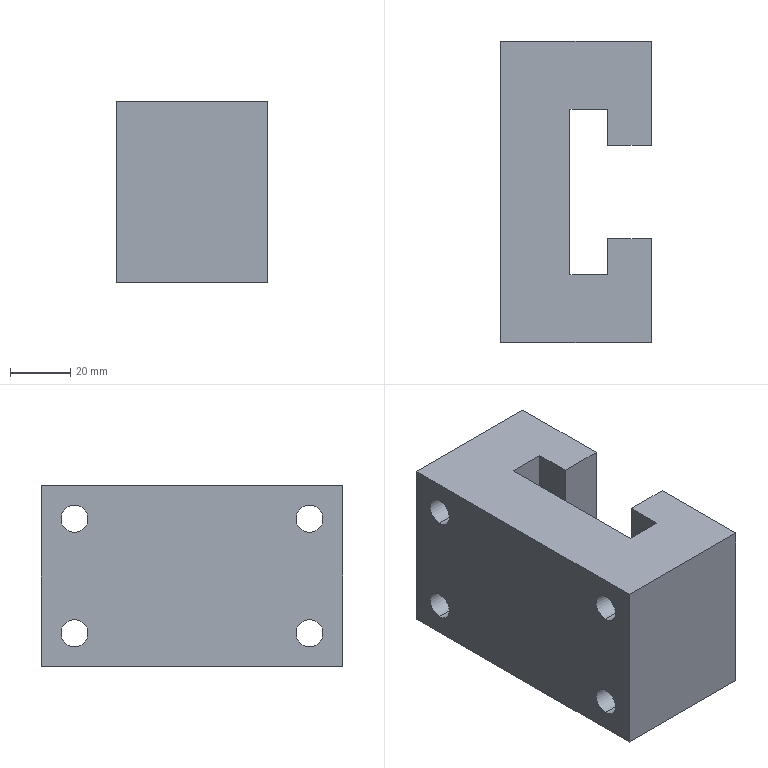Component | SolidWorks | ZN-A-019-1 | 1 solid | 34 faces | box 50 x 100 x 60 mm | volume 215166 mm3 | plane 18 | cylinder 16 | commonest cylinder face diameters 15 x8 9 x8
build123d program:
from build123d import *

# Parameters (mm, degrees)
SKETCH1_W                                       = 100
SKETCH1_H                                       = 50
BOSS_EXTRUDE1_DEPTH                             = 60
CUT_EXTRUDE1_DEPTH                              = 83.006
M8_HEX_SOCKET_HEAD_CAP_SCREW_CBORE1_D           = 9
M8_HEX_SOCKET_HEAD_CAP_SCREW_CBORE1_CBORE_D     = 15
M8_HEX_SOCKET_HEAD_CAP_SCREW_CBORE1_CBORE_DEPTH = 8.6


with BuildPart() as part:
    # Sketch1 → Boss-Extrude1 (new body)
    with BuildSketch(Plane.XY):
        Rectangle(SKETCH1_W, SKETCH1_H)
    extrude(amount=BOSS_EXTRUDE1_DEPTH)

    # Sketch2 → Cut-Extrude1 (cut, through all)
    with BuildSketch(Plane(origin=(0, 0, 0), x_dir=(-1, 0, 0), z_dir=(0, 0, -1))):
        Polygon((-15.5, 25), (15.5, 25), (15.5, 10.5), (27.5, 10.5), (27.5, -2), (-27.5, -2), (-27.5, 10.5), (-15.5, 10.5), align=None)
    extrude(amount=-CUT_EXTRUDE1_DEPTH, mode=Mode.SUBTRACT)

    # M8 Hex Socket Head Cap Screw CBORE1 (through all)
    with Locations(Plane(origin=(0, 25, 0), x_dir=(1, 0, 0), z_dir=(0, 1, 0))):
        with Locations((-39, -11), (-39, -49), (39, -11), (39, -49)):
            CounterBoreHole(M8_HEX_SOCKET_HEAD_CAP_SCREW_CBORE1_D / 2, M8_HEX_SOCKET_HEAD_CAP_SCREW_CBORE1_CBORE_D / 2, M8_HEX_SOCKET_HEAD_CAP_SCREW_CBORE1_CBORE_DEPTH)


solid = part.part

# Placed as in the assembly
solid = solid.moved(Location((540.892, 232.499, 73), (0, 0, -90)))
STEP:
#1=COLOUR_RGB('',0.7922,0.8196,0.9333);
#2=FILL_AREA_STYLE_COLOUR('',#1);
#3=FILL_AREA_STYLE('',(#2));
#4=SURFACE_STYLE_FILL_AREA(#3);
#5=SURFACE_SIDE_STYLE('',(#4));
#6=SURFACE_STYLE_USAGE(.BOTH.,#5);
#7=PRESENTATION_STYLE_ASSIGNMENT((#6));
#8=CARTESIAN_POINT('',(21.941,10.689,3.012));
#9=VERTEX_POINT('',#8);
#10=CARTESIAN_POINT('',(21.941,10.689,3.602));
#11=VERTEX_POINT('',#10);
#12=CARTESIAN_POINT('',(21.941,10.689,3.307));
#13=DIRECTION('',(1.,-0.,0.));
#14=DIRECTION('',(0.,-0.,1.));
#15=AXIS2_PLACEMENT_3D('',#12,#13,#14);
#16=CIRCLE('',#15,0.2953);
#17=EDGE_CURVE('',#9,#11,#16,.T.);
#18=ORIENTED_EDGE('',*,*,#17,.F.);
#19=CARTESIAN_POINT('',(22.279,10.689,3.012));
#20=VERTEX_POINT('',#19);
#21=CARTESIAN_POINT('',(22.279,10.689,3.012));
#22=DIRECTION('',(1.,-0.,0.));
#23=VECTOR('',#22,39.37);
#24=LINE('',#21,#23);
#25=EDGE_CURVE('',#9,#20,#24,.T.);
#26=ORIENTED_EDGE('',*,*,#25,.T.);
#27=CARTESIAN_POINT('',(22.279,10.689,3.602));
#28=VERTEX_POINT('',#27);
#29=CARTESIAN_POINT('',(22.279,10.689,3.307));
#30=DIRECTION('',(1.,-0.,0.));
#31=DIRECTION('',(0.,-0.,1.));
#32=AXIS2_PLACEMENT_3D('',#29,#30,#31);
#33=CIRCLE('',#32,0.2953);
#34=EDGE_CURVE('',#20,#28,#33,.T.);
#35=ORIENTED_EDGE('',*,*,#34,.T.);
#36=CARTESIAN_POINT('',(22.279,10.689,3.602));
#37=DIRECTION('',(1.,-0.,0.));
#38=VECTOR('',#37,39.37);
#39=LINE('',#36,#38);
#40=EDGE_CURVE('',#11,#28,#39,.T.);
#41=ORIENTED_EDGE('',*,*,#40,.F.);
#42=EDGE_LOOP('',(#18,#26,#35,#41));
#43=FACE_OUTER_BOUND('',#42,.T.);
#44=CARTESIAN_POINT('',(22.279,10.689,3.307));
#45=DIRECTION('',(1.,-0.,0.));
#46=DIRECTION('',(0.,-0.,1.));
#47=AXIS2_PLACEMENT_3D('',#44,#45,#46);
#48=CYLINDRICAL_SURFACE('',#47,0.2953);
#49=ADVANCED_FACE('',(#43),#48,.F.);
#50=CARTESIAN_POINT('',(20.311,10.689,3.13));
#51=VERTEX_POINT('',#50);
#52=CARTESIAN_POINT('',(20.311,10.689,3.484));
#53=VERTEX_POINT('',#52);
#54=CARTESIAN_POINT('',(20.311,10.689,3.307));
#55=DIRECTION('',(1.,-0.,0.));
#56=DIRECTION('',(0.,-0.,1.));
#57=AXIS2_PLACEMENT_3D('',#54,#55,#56);
#58=CIRCLE('',#57,0.1772);
#59=EDGE_CURVE('',#51,#53,#58,.T.);
#60=ORIENTED_EDGE('',*,*,#59,.F.);
#61=CARTESIAN_POINT('',(21.941,10.689,3.13));
#62=VERTEX_POINT('',#61);
#63=CARTESIAN_POINT('',(22.279,10.689,3.13));
#64=DIRECTION('',(1.,-0.,0.));
#65=VECTOR('',#64,39.37);
#66=LINE('',#63,#65);
#67=EDGE_CURVE('',#51,#62,#66,.T.);
#68=ORIENTED_EDGE('',*,*,#67,.T.);
#69=CARTESIAN_POINT('',(21.941,10.689,3.484));
#70=VERTEX_POINT('',#69);
#71=CARTESIAN_POINT('',(21.941,10.689,3.307));
#72=DIRECTION('',(1.,-0.,0.));
#73=DIRECTION('',(0.,-0.,1.));
#74=AXIS2_PLACEMENT_3D('',#71,#72,#73);
#75=CIRCLE('',#74,0.1772);
#76=EDGE_CURVE('',#62,#70,#75,.T.);
#77=ORIENTED_EDGE('',*,*,#76,.T.);
#78=CARTESIAN_POINT('',(22.279,10.689,3.484));
#79=DIRECTION('',(1.,-0.,0.));
#80=VECTOR('',#79,39.37);
#81=LINE('',#78,#80);
#82=EDGE_CURVE('',#53,#70,#81,.T.);
#83=ORIENTED_EDGE('',*,*,#82,.F.);
#84=EDGE_LOOP('',(#60,#68,#77,#83));
#85=FACE_OUTER_BOUND('',#84,.T.);
#86=CARTESIAN_POINT('',(22.279,10.689,3.307));
#87=DIRECTION('',(1.,-0.,0.));
#88=DIRECTION('',(0.,-0.,1.));
#89=AXIS2_PLACEMENT_3D('',#86,#87,#88);
#90=CYLINDRICAL_SURFACE('',#89,0.1772);
#91=ADVANCED_FACE('',(#85),#90,.F.);
#92=CARTESIAN_POINT('',(21.941,10.689,4.508));
#93=VERTEX_POINT('',#92);
#94=CARTESIAN_POINT('',(21.941,10.689,5.098));
#95=VERTEX_POINT('',#94);
#96=CARTESIAN_POINT('',(21.941,10.689,4.803));
#97=DIRECTION('',(1.,-0.,0.));
#98=DIRECTION('',(0.,-0.,1.));
#99=AXIS2_PLACEMENT_3D('',#96,#97,#98);
#100=CIRCLE('',#99,0.2953);
#101=EDGE_CURVE('',#93,#95,#100,.T.);
#102=ORIENTED_EDGE('',*,*,#101,.F.);
#103=CARTESIAN_POINT('',(22.279,10.689,4.508));
#104=VERTEX_POINT('',#103);
#105=CARTESIAN_POINT('',(22.279,10.689,4.508));
#106=DIRECTION('',(1.,-0.,0.));
#107=VECTOR('',#106,39.37);
#108=LINE('',#105,#107);
#109=EDGE_CURVE('',#93,#104,#108,.T.);
#110=ORIENTED_EDGE('',*,*,#109,.T.);
#111=CARTESIAN_POINT('',(22.279,10.689,5.098));
#112=VERTEX_POINT('',#111);
#113=CARTESIAN_POINT('',(22.279,10.689,4.803));
#114=DIRECTION('',(1.,-0.,0.));
#115=DIRECTION('',(0.,-0.,1.));
#116=AXIS2_PLACEMENT_3D('',#113,#114,#115);
#117=CIRCLE('',#116,0.2953);
#118=EDGE_CURVE('',#104,#112,#117,.T.);
#119=ORIENTED_EDGE('',*,*,#118,.T.);
#120=CARTESIAN_POINT('',(22.279,10.689,5.098));
#121=DIRECTION('',(1.,-0.,0.));
#122=VECTOR('',#121,39.37);
#123=LINE('',#120,#122);
#124=EDGE_CURVE('',#95,#112,#123,.T.);
#125=ORIENTED_EDGE('',*,*,#124,.F.);
#126=EDGE_LOOP('',(#102,#110,#119,#125));
#127=FACE_OUTER_BOUND('',#126,.T.);
#128=CARTESIAN_POINT('',(22.279,10.689,4.803));
#129=DIRECTION('',(1.,-0.,0.));
#130=DIRECTION('',(0.,-0.,1.));
#131=AXIS2_PLACEMENT_3D('',#128,#129,#130);
#132=CYLINDRICAL_SURFACE('',#131,0.2953);
#133=ADVANCED_FACE('',(#127),#132,.F.);
#134=CARTESIAN_POINT('',(20.311,10.689,4.626));
#135=VERTEX_POINT('',#134);
#136=CARTESIAN_POINT('',(20.311,10.689,4.98));
#137=VERTEX_POINT('',#136);
#138=CARTESIAN_POINT('',(20.311,10.689,4.803));
#139=DIRECTION('',(1.,-0.,0.));
#140=DIRECTION('',(0.,-0.,1.));
#141=AXIS2_PLACEMENT_3D('',#138,#139,#140);
#142=CIRCLE('',#141,0.1772);
#143=EDGE_CURVE('',#135,#137,#142,.T.);
#144=ORIENTED_EDGE('',*,*,#143,.F.);
#145=CARTESIAN_POINT('',(21.941,10.689,4.626));
#146=VERTEX_POINT('',#145);
#147=CARTESIAN_POINT('',(22.279,10.689,4.626));
#148=DIRECTION('',(1.,-0.,0.));
#149=VECTOR('',#148,39.37);
#150=LINE('',#147,#149);
#151=EDGE_CURVE('',#135,#146,#150,.T.);
#152=ORIENTED_EDGE('',*,*,#151,.T.);
#153=CARTESIAN_POINT('',(21.941,10.689,4.98));
#154=VERTEX_POINT('',#153);
#155=CARTESIAN_POINT('',(21.941,10.689,4.803));
#156=DIRECTION('',(1.,-0.,0.));
#157=DIRECTION('',(0.,-0.,1.));
#158=AXIS2_PLACEMENT_3D('',#155,#156,#157);
#159=CIRCLE('',#158,0.1772);
#160=EDGE_CURVE('',#146,#154,#159,.T.);
#161=ORIENTED_EDGE('',*,*,#160,.T.);
#162=CARTESIAN_POINT('',(22.279,10.689,4.98));
#163=DIRECTION('',(1.,-0.,0.));
#164=VECTOR('',#163,39.37);
#165=LINE('',#162,#164);
#166=EDGE_CURVE('',#137,#154,#165,.T.);
#167=ORIENTED_EDGE('',*,*,#166,.F.);
#168=EDGE_LOOP('',(#144,#152,#161,#167));
#169=FACE_OUTER_BOUND('',#168,.T.);
#170=CARTESIAN_POINT('',(22.279,10.689,4.803));
#171=DIRECTION('',(1.,-0.,0.));
#172=DIRECTION('',(0.,-0.,1.));
#173=AXIS2_PLACEMENT_3D('',#170,#171,#172);
#174=CYLINDRICAL_SURFACE('',#173,0.1772);
#175=ADVANCED_FACE('',(#169),#174,.F.);
#176=CARTESIAN_POINT('',(21.941,7.618,3.012));
#177=VERTEX_POINT('',#176);
#178=CARTESIAN_POINT('',(21.941,7.618,3.602));
#179=VERTEX_POINT('',#178);
#180=CARTESIAN_POINT('',(21.941,7.618,3.307));
#181=DIRECTION('',(1.,-0.,0.));
#182=DIRECTION('',(0.,-0.,1.));
#183=AXIS2_PLACEMENT_3D('',#180,#181,#182);
#184=CIRCLE('',#183,0.2953);
#185=EDGE_CURVE('',#177,#179,#184,.T.);
#186=ORIENTED_EDGE('',*,*,#185,.F.);
#187=CARTESIAN_POINT('',(22.279,7.618,3.012));
#188=VERTEX_POINT('',#187);
#189=CARTESIAN_POINT('',(22.279,7.618,3.012));
#190=DIRECTION('',(1.,-0.,0.));
#191=VECTOR('',#190,39.37);
#192=LINE('',#189,#191);
#193=EDGE_CURVE('',#177,#188,#192,.T.);
#194=ORIENTED_EDGE('',*,*,#193,.T.);
#195=CARTESIAN_POINT('',(22.279,7.618,3.602));
#196=VERTEX_POINT('',#195);
#197=CARTESIAN_POINT('',(22.279,7.618,3.307));
#198=DIRECTION('',(1.,-0.,0.));
#199=DIRECTION('',(0.,-0.,1.));
#200=AXIS2_PLACEMENT_3D('',#197,#198,#199);
#201=CIRCLE('',#200,0.2953);
#202=EDGE_CURVE('',#188,#196,#201,.T.);
#203=ORIENTED_EDGE('',*,*,#202,.T.);
#204=CARTESIAN_POINT('',(22.279,7.618,3.602));
#205=DIRECTION('',(1.,-0.,0.));
#206=VECTOR('',#205,39.37);
#207=LINE('',#204,#206);
#208=EDGE_CURVE('',#179,#196,#207,.T.);
#209=ORIENTED_EDGE('',*,*,#208,.F.);
#210=EDGE_LOOP('',(#186,#194,#203,#209));
#211=FACE_OUTER_BOUND('',#210,.T.);
#212=CARTESIAN_POINT('',(22.279,7.618,3.307));
#213=DIRECTION('',(1.,-0.,0.));
#214=DIRECTION('',(0.,-0.,1.));
#215=AXIS2_PLACEMENT_3D('',#212,#213,#214);
#216=CYLINDRICAL_SURFACE('',#215,0.2953);
#217=ADVANCED_FACE('',(#211),#216,.F.);
#218=CARTESIAN_POINT('',(20.311,7.618,3.13));
#219=VERTEX_POINT('',#218);
#220=CARTESIAN_POINT('',(20.311,7.618,3.484));
#221=VERTEX_POINT('',#220);
#222=CARTESIAN_POINT('',(20.311,7.618,3.307));
#223=DIRECTION('',(1.,-0.,0.));
#224=DIRECTION('',(0.,-0.,1.));
#225=AXIS2_PLACEMENT_3D('',#222,#223,#224);
#226=CIRCLE('',#225,0.1772);
#227=EDGE_CURVE('',#219,#221,#226,.T.);
#228=ORIENTED_EDGE('',*,*,#227,.F.);
#229=CARTESIAN_POINT('',(21.941,7.618,3.13));
#230=VERTEX_POINT('',#229);
#231=CARTESIAN_POINT('',(22.279,7.618,3.13));
#232=DIRECTION('',(1.,-0.,0.));
#233=VECTOR('',#232,39.37);
#234=LINE('',#231,#233);
#235=EDGE_CURVE('',#219,#230,#234,.T.);
#236=ORIENTED_EDGE('',*,*,#235,.T.);
#237=CARTESIAN_POINT('',(21.941,7.618,3.484));
#238=VERTEX_POINT('',#237);
#239=CARTESIAN_POINT('',(21.941,7.618,3.307));
#240=DIRECTION('',(1.,-0.,0.));
#241=DIRECTION('',(0.,-0.,1.));
#242=AXIS2_PLACEMENT_3D('',#239,#240,#241);
#243=CIRCLE('',#242,0.1772);
#244=EDGE_CURVE('',#230,#238,#243,.T.);
#245=ORIENTED_EDGE('',*,*,#244,.T.);
#246=CARTESIAN_POINT('',(22.279,7.618,3.484));
#247=DIRECTION('',(1.,-0.,0.));
#248=VECTOR('',#247,39.37);
#249=LINE('',#246,#248);
#250=EDGE_CURVE('',#221,#238,#249,.T.);
#251=ORIENTED_EDGE('',*,*,#250,.F.);
#252=EDGE_LOOP('',(#228,#236,#245,#251));
#253=FACE_OUTER_BOUND('',#252,.T.);
#254=CARTESIAN_POINT('',(22.279,7.618,3.307));
#255=DIRECTION('',(1.,-0.,0.));
#256=DIRECTION('',(0.,-0.,1.));
#257=AXIS2_PLACEMENT_3D('',#254,#255,#256);
#258=CYLINDRICAL_SURFACE('',#257,0.1772);
#259=ADVANCED_FACE('',(#253),#258,.F.);
#260=CARTESIAN_POINT('',(21.941,7.618,4.508));
#261=VERTEX_POINT('',#260);
#262=CARTESIAN_POINT('',(21.941,7.618,5.098));
#263=VERTEX_POINT('',#262);
#264=CARTESIAN_POINT('',(21.941,7.618,4.803));
#265=DIRECTION('',(1.,-0.,0.));
#266=DIRECTION('',(0.,-0.,1.));
#267=AXIS2_PLACEMENT_3D('',#264,#265,#266);
#268=CIRCLE('',#267,0.2953);
#269=EDGE_CURVE('',#261,#263,#268,.T.);
#270=ORIENTED_EDGE('',*,*,#269,.F.);
#271=CARTESIAN_POINT('',(22.279,7.618,4.508));
#272=VERTEX_POINT('',#271);
#273=CARTESIAN_POINT('',(22.279,7.618,4.508));
#274=DIRECTION('',(1.,-0.,0.));
#275=VECTOR('',#274,39.37);
#276=LINE('',#273,#275);
#277=EDGE_CURVE('',#261,#272,#276,.T.);
#278=ORIENTED_EDGE('',*,*,#277,.T.);
#279=CARTESIAN_POINT('',(22.279,7.618,5.098));
#280=VERTEX_POINT('',#279);
#281=CARTESIAN_POINT('',(22.279,7.618,4.803));
#282=DIRECTION('',(1.,-0.,0.));
#283=DIRECTION('',(0.,-0.,1.));
#284=AXIS2_PLACEMENT_3D('',#281,#282,#283);
#285=CIRCLE('',#284,0.2953);
#286=EDGE_CURVE('',#272,#280,#285,.T.);
#287=ORIENTED_EDGE('',*,*,#286,.T.);
#288=CARTESIAN_POINT('',(22.279,7.618,5.098));
#289=DIRECTION('',(1.,-0.,0.));
#290=VECTOR('',#289,39.37);
#291=LINE('',#288,#290);
#292=EDGE_CURVE('',#263,#280,#291,.T.);
#293=ORIENTED_EDGE('',*,*,#292,.F.);
#294=EDGE_LOOP('',(#270,#278,#287,#293));
#295=FACE_OUTER_BOUND('',#294,.T.);
#296=CARTESIAN_POINT('',(22.279,7.618,4.803));
#297=DIRECTION('',(1.,-0.,0.));
#298=DIRECTION('',(0.,-0.,1.));
#299=AXIS2_PLACEMENT_3D('',#296,#297,#298);
#300=CYLINDRICAL_SURFACE('',#299,0.2953);
#301=ADVANCED_FACE('',(#295),#300,.F.);
#302=CARTESIAN_POINT('',(20.311,7.618,4.626));
#303=VERTEX_POINT('',#302);
#304=CARTESIAN_POINT('',(20.311,7.618,4.98));
#305=VERTEX_POINT('',#304);
#306=CARTESIAN_POINT('',(20.311,7.618,4.803));
#307=DIRECTION('',(1.,-0.,0.));
#308=DIRECTION('',(0.,-0.,1.));
#309=AXIS2_PLACEMENT_3D('',#306,#307,#308);
#310=CIRCLE('',#309,0.1772);
#311=EDGE_CURVE('',#303,#305,#310,.T.);
#312=ORIENTED_EDGE('',*,*,#311,.F.);
#313=CARTESIAN_POINT('',(21.941,7.618,4.626));
#314=VERTEX_POINT('',#313);
#315=CARTESIAN_POINT('',(22.279,7.618,4.626));
#316=DIRECTION('',(1.,-0.,0.));
#317=VECTOR('',#316,39.37);
#318=LINE('',#315,#317);
#319=EDGE_CURVE('',#303,#314,#318,.T.);
#320=ORIENTED_EDGE('',*,*,#319,.T.);
#321=CARTESIAN_POINT('',(21.941,7.618,4.98));
#322=VERTEX_POINT('',#321);
#323=CARTESIAN_POINT('',(21.941,7.618,4.803));
#324=DIRECTION('',(1.,-0.,0.));
#325=DIRECTION('',(0.,-0.,1.));
#326=AXIS2_PLACEMENT_3D('',#323,#324,#325);
#327=CIRCLE('',#326,0.1772);
#328=EDGE_CURVE('',#314,#322,#327,.T.);
#329=ORIENTED_EDGE('',*,*,#328,.T.);
#330=CARTESIAN_POINT('',(22.279,7.618,4.98));
#331=DIRECTION('',(1.,-0.,0.));
#332=VECTOR('',#331,39.37);
#333=LINE('',#330,#332);
#334=EDGE_CURVE('',#305,#322,#333,.T.);
#335=ORIENTED_EDGE('',*,*,#334,.F.);
#336=EDGE_LOOP('',(#312,#320,#329,#335));
#337=FACE_OUTER_BOUND('',#336,.T.);
#338=CARTESIAN_POINT('',(22.279,7.618,4.803));
#339=DIRECTION('',(1.,-0.,0.));
#340=DIRECTION('',(0.,-0.,1.));
#341=AXIS2_PLACEMENT_3D('',#338,#339,#340);
#342=CYLINDRICAL_SURFACE('',#341,0.1772);
#343=ADVANCED_FACE('',(#337),#342,.F.);
#344=CARTESIAN_POINT('',(22.279,7.618,3.307));
#345=DIRECTION('',(1.,-0.,0.));
#346=DIRECTION('',(0.,-0.,1.));
#347=AXIS2_PLACEMENT_3D('',#344,#345,#346);
#348=CIRCLE('',#347,0.2953);
#349=EDGE_CURVE('',#196,#188,#348,.T.);
#350=ORIENTED_EDGE('',*,*,#349,.F.);
#351=ORIENTED_EDGE('',*,*,#202,.F.);
#352=EDGE_LOOP('',(#350,#351));
#353=FACE_BOUND('',#352,.T.);
#354=CARTESIAN_POINT('',(22.279,7.618,4.803));
#355=DIRECTION('',(1.,-0.,0.));
#356=DIRECTION('',(0.,-0.,1.));
#357=AXIS2_PLACEMENT_3D('',#354,#355,#356);
#358=CIRCLE('',#357,0.2953);
#359=EDGE_CURVE('',#280,#272,#358,.T.);
#360=ORIENTED_EDGE('',*,*,#359,.F.);
#361=ORIENTED_EDGE('',*,*,#286,.F.);
#362=EDGE_LOOP('',(#360,#361));
#363=FACE_BOUND('',#362,.T.);
#364=CARTESIAN_POINT('',(22.279,7.185,2.874));
#365=VERTEX_POINT('',#364);
#366=CARTESIAN_POINT('',(22.279,8.543,2.874));
#367=VERTEX_POINT('',#366);
#368=CARTESIAN_POINT('',(22.279,11.122,2.874));
#369=DIRECTION('',(0.,1.,0.));
#370=VECTOR('',#369,39.37);
#371=LINE('',#368,#370);
#372=EDGE_CURVE('',#365,#367,#371,.T.);
#373=ORIENTED_EDGE('',*,*,#372,.T.);
#374=CARTESIAN_POINT('',(22.279,8.543,5.236));
#375=VERTEX_POINT('',#374);
#376=CARTESIAN_POINT('',(22.279,8.543,5.236));
#377=DIRECTION('',(0.,0.,-1.));
#378=VECTOR('',#377,39.37);
#379=LINE('',#376,#378);
#380=EDGE_CURVE('',#375,#367,#379,.T.);
#381=ORIENTED_EDGE('',*,*,#380,.F.);
#382=CARTESIAN_POINT('',(22.279,7.185,5.236));
#383=VERTEX_POINT('',#382);
#384=CARTESIAN_POINT('',(22.279,11.122,5.236));
#385=DIRECTION('',(0.,1.,0.));
#386=VECTOR('',#385,39.37);
#387=LINE('',#384,#386);
#388=EDGE_CURVE('',#383,#375,#387,.T.);
#389=ORIENTED_EDGE('',*,*,#388,.F.);
#390=CARTESIAN_POINT('',(22.279,7.185,5.236));
#391=DIRECTION('',(0.,0.,-1.));
#392=VECTOR('',#391,39.37);
#393=LINE('',#390,#392);
#394=EDGE_CURVE('',#383,#365,#393,.T.);
#395=ORIENTED_EDGE('',*,*,#394,.T.);
#396=EDGE_LOOP('',(#373,#381,#389,#395));
#397=FACE_OUTER_BOUND('',#396,.T.);
#398=CARTESIAN_POINT('',(22.279,11.122,5.236));
#399=DIRECTION('',(-1.,0.,-0.));
#400=DIRECTION('',(0.,0.,-1.));
#401=AXIS2_PLACEMENT_3D('',#398,#399,#400);
#402=PLANE('',#401);
#403=ADVANCED_FACE('',(#353,#363,#397),#402,.F.);
#404=CARTESIAN_POINT('',(20.311,7.185,2.874));
#405=VERTEX_POINT('',#404);
#406=CARTESIAN_POINT('',(20.311,7.185,2.874));
#407=DIRECTION('',(1.,-0.,0.));
#408=VECTOR('',#407,39.37);
#409=LINE('',#406,#408);
#410=EDGE_CURVE('',#405,#365,#409,.T.);
#411=ORIENTED_EDGE('',*,*,#410,.T.);
#412=ORIENTED_EDGE('',*,*,#394,.F.);
#413=CARTESIAN_POINT('',(20.311,7.185,5.236));
#414=VERTEX_POINT('',#413);
#415=CARTESIAN_POINT('',(20.311,7.185,5.236));
#416=DIRECTION('',(1.,-0.,0.));
#417=VECTOR('',#416,39.37);
#418=LINE('',#415,#417);
#419=EDGE_CURVE('',#414,#383,#418,.T.);
#420=ORIENTED_EDGE('',*,*,#419,.F.);
#421=CARTESIAN_POINT('',(20.311,7.185,5.236));
#422=DIRECTION('',(0.,0.,-1.));
#423=VECTOR('',#422,39.37);
#424=LINE('',#421,#423);
#425=EDGE_CURVE('',#414,#405,#424,.T.);
#426=ORIENTED_EDGE('',*,*,#425,.T.);
#427=EDGE_LOOP('',(#411,#412,#420,#426));
#428=FACE_OUTER_BOUND('',#427,.T.);
#429=CARTESIAN_POINT('',(20.311,7.185,5.236));
#430=DIRECTION('',(0.,1.,0.));
#431=DIRECTION('',(-0.,-0.,1.));
#432=AXIS2_PLACEMENT_3D('',#429,#430,#431);
#433=PLANE('',#432);
#434=ADVANCED_FACE('',(#428),#433,.F.);
#435=CARTESIAN_POINT('',(22.279,10.689,3.307));
#436=DIRECTION('',(1.,-0.,0.));
#437=DIRECTION('',(0.,-0.,1.));
#438=AXIS2_PLACEMENT_3D('',#435,#436,#437);
#439=CIRCLE('',#438,0.2953);
#440=EDGE_CURVE('',#28,#20,#439,.T.);
#441=ORIENTED_EDGE('',*,*,#440,.F.);
#442=ORIENTED_EDGE('',*,*,#34,.F.);
#443=EDGE_LOOP('',(#441,#442));
#444=FACE_BOUND('',#443,.T.);
#445=CARTESIAN_POINT('',(22.279,10.689,4.803));
#446=DIRECTION('',(1.,-0.,0.));
#447=DIRECTION('',(0.,-0.,1.));
#448=AXIS2_PLACEMENT_3D('',#445,#446,#447);
#449=CIRCLE('',#448,0.2953);
#450=EDGE_CURVE('',#112,#104,#449,.T.);
#451=ORIENTED_EDGE('',*,*,#450,.F.);
#452=ORIENTED_EDGE('',*,*,#118,.F.);
#453=EDGE_LOOP('',(#451,#452));
#454=FACE_BOUND('',#453,.T.);
#455=CARTESIAN_POINT('',(22.279,9.764,5.236));
#456=VERTEX_POINT('',#455);
#457=CARTESIAN_POINT('',(22.279,11.122,5.236));
#458=VERTEX_POINT('',#457);
#459=CARTESIAN_POINT('',(22.279,11.122,5.236));
#460=DIRECTION('',(0.,1.,0.));
#461=VECTOR('',#460,39.37);
#462=LINE('',#459,#461);
#463=EDGE_CURVE('',#456,#458,#462,.T.);
#464=ORIENTED_EDGE('',*,*,#463,.F.);
#465=CARTESIAN_POINT('',(22.279,9.764,2.874));
#466=VERTEX_POINT('',#465);
#467=CARTESIAN_POINT('',(22.279,9.764,5.236));
#468=DIRECTION('',(0.,0.,-1.));
#469=VECTOR('',#468,39.37);
#470=LINE('',#467,#469);
#471=EDGE_CURVE('',#456,#466,#470,.T.);
#472=ORIENTED_EDGE('',*,*,#471,.T.);
#473=CARTESIAN_POINT('',(22.279,11.122,2.874));
#474=VERTEX_POINT('',#473);
#475=CARTESIAN_POINT('',(22.279,11.122,2.874));
#476=DIRECTION('',(0.,1.,0.));
#477=VECTOR('',#476,39.37);
#478=LINE('',#475,#477);
#479=EDGE_CURVE('',#466,#474,#478,.T.);
#480=ORIENTED_EDGE('',*,*,#479,.T.);
#481=CARTESIAN_POINT('',(22.279,11.122,5.236));
#482=DIRECTION('',(0.,0.,-1.));
#483=VECTOR('',#482,39.37);
#484=LINE('',#481,#483);
#485=EDGE_CURVE('',#458,#474,#484,.T.);
#486=ORIENTED_EDGE('',*,*,#485,.F.);
#487=EDGE_LOOP('',(#464,#472,#480,#486));
#488=FACE_OUTER_BOUND('',#487,.T.);
#489=CARTESIAN_POINT('',(22.279,11.122,5.236));
#490=DIRECTION('',(-1.,0.,-0.));
#491=DIRECTION('',(0.,0.,-1.));
#492=AXIS2_PLACEMENT_3D('',#489,#490,#491);
#493=PLANE('',#492);
#494=ADVANCED_FACE('',(#444,#454,#488),#493,.F.);
#495=CARTESIAN_POINT('',(20.311,11.122,2.874));
#496=VERTEX_POINT('',#495);
#497=CARTESIAN_POINT('',(20.311,11.122,2.874));
#498=DIRECTION('',(-1.,0.,-0.));
#499=VECTOR('',#498,39.37);
#500=LINE('',#497,#499);
#501=EDGE_CURVE('',#474,#496,#500,.T.);
#502=ORIENTED_EDGE('',*,*,#501,.T.);
#503=CARTESIAN_POINT('',(20.311,11.122,5.236));
#504=VERTEX_POINT('',#503);
#505=CARTESIAN_POINT('',(20.311,11.122,5.236));
#506=DIRECTION('',(0.,0.,-1.));
#507=VECTOR('',#506,39.37);
#508=LINE('',#505,#507);
#509=EDGE_CURVE('',#504,#496,#508,.T.);
#510=ORIENTED_EDGE('',*,*,#509,.F.);
#511=CARTESIAN_POINT('',(20.311,11.122,5.236));
#512=DIRECTION('',(-1.,0.,-0.));
#513=VECTOR('',#512,39.37);
#514=LINE('',#511,#513);
#515=EDGE_CURVE('',#458,#504,#514,.T.);
#516=ORIENTED_EDGE('',*,*,#515,.F.);
#517=ORIENTED_EDGE('',*,*,#485,.T.);
#518=EDGE_LOOP('',(#502,#510,#516,#517));
#519=FACE_OUTER_BOUND('',#518,.T.);
#520=CARTESIAN_POINT('',(20.311,11.122,5.236));
#521=DIRECTION('',(-0.,-1.,-0.));
#522=DIRECTION('',(0.,0.,-1.));
#523=AXIS2_PLACEMENT_3D('',#520,#521,#522);
#524=PLANE('',#523);
#525=ADVANCED_FACE('',(#519),#524,.F.);
#526=CARTESIAN_POINT('',(20.311,10.689,3.307));
#527=DIRECTION('',(1.,-0.,0.));
#528=DIRECTION('',(0.,-0.,1.));
#529=AXIS2_PLACEMENT_3D('',#526,#527,#528);
#530=CIRCLE('',#529,0.1772);
#531=EDGE_CURVE('',#53,#51,#530,.T.);
#532=ORIENTED_EDGE('',*,*,#531,.T.);
#533=ORIENTED_EDGE('',*,*,#59,.T.);
#534=EDGE_LOOP('',(#532,#533));
#535=FACE_BOUND('',#534,.T.);
#536=CARTESIAN_POINT('',(20.311,10.689,4.803));
#537=DIRECTION('',(1.,-0.,0.));
#538=DIRECTION('',(0.,-0.,1.));
#539=AXIS2_PLACEMENT_3D('',#536,#537,#538);
#540=CIRCLE('',#539,0.1772);
#541=EDGE_CURVE('',#137,#135,#540,.T.);
#542=ORIENTED_EDGE('',*,*,#541,.T.);
#543=ORIENTED_EDGE('',*,*,#143,.T.);
#544=EDGE_LOOP('',(#542,#543));
#545=FACE_BOUND('',#544,.T.);
#546=CARTESIAN_POINT('',(20.311,7.618,3.307));
#547=DIRECTION('',(1.,-0.,0.));
#548=DIRECTION('',(0.,-0.,1.));
#549=AXIS2_PLACEMENT_3D('',#546,#547,#548);
#550=CIRCLE('',#549,0.1772);
#551=EDGE_CURVE('',#221,#219,#550,.T.);
#552=ORIENTED_EDGE('',*,*,#551,.T.);
#553=ORIENTED_EDGE('',*,*,#227,.T.);
#554=EDGE_LOOP('',(#552,#553));
#555=FACE_BOUND('',#554,.T.);
#556=CARTESIAN_POINT('',(20.311,7.618,4.803));
#557=DIRECTION('',(1.,-0.,0.));
#558=DIRECTION('',(0.,-0.,1.));
#559=AXIS2_PLACEMENT_3D('',#556,#557,#558);
#560=CIRCLE('',#559,0.1772);
#561=EDGE_CURVE('',#305,#303,#560,.T.);
#562=ORIENTED_EDGE('',*,*,#561,.T.);
#563=ORIENTED_EDGE('',*,*,#311,.T.);
#564=EDGE_LOOP('',(#562,#563));
#565=FACE_BOUND('',#564,.T.);
#566=CARTESIAN_POINT('',(20.311,11.122,2.874));
#567=DIRECTION('',(-0.,-1.,-0.));
#568=VECTOR('',#567,39.37);
#569=LINE('',#566,#568);
#570=EDGE_CURVE('',#496,#405,#569,.T.);
#571=ORIENTED_EDGE('',*,*,#570,.T.);
#572=ORIENTED_EDGE('',*,*,#425,.F.);
#573=CARTESIAN_POINT('',(20.311,11.122,5.236));
#574=DIRECTION('',(-0.,-1.,-0.));
#575=VECTOR('',#574,39.37);
#576=LINE('',#573,#575);
#577=EDGE_CURVE('',#504,#414,#576,.T.);
#578=ORIENTED_EDGE('',*,*,#577,.F.);
#579=ORIENTED_EDGE('',*,*,#509,.T.);
#580=EDGE_LOOP('',(#571,#572,#578,#579));
#581=FACE_OUTER_BOUND('',#580,.T.);
#582=CARTESIAN_POINT('',(20.311,11.122,5.236));
#583=DIRECTION('',(1.,-0.,0.));
#584=DIRECTION('',(-0.,-0.,1.));
#585=AXIS2_PLACEMENT_3D('',#582,#583,#584);
#586=PLANE('',#585);
#587=ADVANCED_FACE('',(#535,#545,#555,#565,#581),#586,.F.);
#588=ORIENTED_EDGE('',*,*,#388,.T.);
#589=CARTESIAN_POINT('',(21.708,8.543,5.236));
#590=VERTEX_POINT('',#589);
#591=CARTESIAN_POINT('',(22.279,8.543,5.236));
#592=DIRECTION('',(-1.,0.,-0.));
#593=VECTOR('',#592,39.37);
#594=LINE('',#591,#593);
#595=EDGE_CURVE('',#375,#590,#594,.T.);
#596=ORIENTED_EDGE('',*,*,#595,.T.);
#597=CARTESIAN_POINT('',(21.708,8.071,5.236));
#598=VERTEX_POINT('',#597);
#599=CARTESIAN_POINT('',(21.708,8.543,5.236));
#600=DIRECTION('',(-0.,-1.,-0.));
#601=VECTOR('',#600,39.37);
#602=LINE('',#599,#601);
#603=EDGE_CURVE('',#590,#598,#602,.T.);
#604=ORIENTED_EDGE('',*,*,#603,.T.);
#605=CARTESIAN_POINT('',(21.216,8.071,5.236));
#606=VERTEX_POINT('',#605);
#607=CARTESIAN_POINT('',(21.708,8.071,5.236));
#608=DIRECTION('',(-1.,0.,-0.));
#609=VECTOR('',#608,39.37);
#610=LINE('',#607,#609);
#611=EDGE_CURVE('',#598,#606,#610,.T.);
#612=ORIENTED_EDGE('',*,*,#611,.T.);
#613=CARTESIAN_POINT('',(21.216,10.236,5.236));
#614=VERTEX_POINT('',#613);
#615=CARTESIAN_POINT('',(21.216,8.071,5.236));
#616=DIRECTION('',(0.,1.,0.));
#617=VECTOR('',#616,39.37);
#618=LINE('',#615,#617);
#619=EDGE_CURVE('',#606,#614,#618,.T.);
#620=ORIENTED_EDGE('',*,*,#619,.T.);
#621=CARTESIAN_POINT('',(21.708,10.236,5.236));
#622=VERTEX_POINT('',#621);
#623=CARTESIAN_POINT('',(21.216,10.236,5.236));
#624=DIRECTION('',(1.,-0.,0.));
#625=VECTOR('',#624,39.37);
#626=LINE('',#623,#625);
#627=EDGE_CURVE('',#614,#622,#626,.T.);
#628=ORIENTED_EDGE('',*,*,#627,.T.);
#629=CARTESIAN_POINT('',(21.708,9.764,5.236));
#630=VERTEX_POINT('',#629);
#631=CARTESIAN_POINT('',(21.708,10.236,5.236));
#632=DIRECTION('',(-0.,-1.,-0.));
#633=VECTOR('',#632,39.37);
#634=LINE('',#631,#633);
#635=EDGE_CURVE('',#622,#630,#634,.T.);
#636=ORIENTED_EDGE('',*,*,#635,.T.);
#637=CARTESIAN_POINT('',(22.279,9.764,5.236));
#638=DIRECTION('',(1.,-0.,0.));
#639=VECTOR('',#638,39.37);
#640=LINE('',#637,#639);
#641=EDGE_CURVE('',#630,#456,#640,.T.);
#642=ORIENTED_EDGE('',*,*,#641,.T.);
#643=ORIENTED_EDGE('',*,*,#463,.T.);
#644=ORIENTED_EDGE('',*,*,#515,.T.);
#645=ORIENTED_EDGE('',*,*,#577,.T.);
#646=ORIENTED_EDGE('',*,*,#419,.T.);
#647=EDGE_LOOP('',(#588,#596,#604,#612,#620,#628,#636,#642,#643,#644,#645,#646));
#648=FACE_OUTER_BOUND('',#647,.T.);
#649=CARTESIAN_POINT('',(21.295,9.154,5.236));
#650=DIRECTION('',(0.,0.,-1.));
#651=DIRECTION('',(0.,1.,0.));
#652=AXIS2_PLACEMENT_3D('',#649,#650,#651);
#653=PLANE('',#652);
#654=ADVANCED_FACE('',(#648),#653,.F.);
#655=CARTESIAN_POINT('',(21.708,8.543,2.874));
#656=VERTEX_POINT('',#655);
#657=CARTESIAN_POINT('',(22.279,8.543,2.874));
#658=DIRECTION('',(-1.,0.,-0.));
#659=VECTOR('',#658,39.37);
#660=LINE('',#657,#659);
#661=EDGE_CURVE('',#367,#656,#660,.T.);
#662=ORIENTED_EDGE('',*,*,#661,.F.);
#663=ORIENTED_EDGE('',*,*,#372,.F.);
#664=ORIENTED_EDGE('',*,*,#410,.F.);
#665=ORIENTED_EDGE('',*,*,#570,.F.);
#666=ORIENTED_EDGE('',*,*,#501,.F.);
#667=ORIENTED_EDGE('',*,*,#479,.F.);
#668=CARTESIAN_POINT('',(21.708,9.764,2.874));
#669=VERTEX_POINT('',#668);
#670=CARTESIAN_POINT('',(22.279,9.764,2.874));
#671=DIRECTION('',(1.,-0.,0.));
#672=VECTOR('',#671,39.37);
#673=LINE('',#670,#672);
#674=EDGE_CURVE('',#669,#466,#673,.T.);
#675=ORIENTED_EDGE('',*,*,#674,.F.);
#676=CARTESIAN_POINT('',(21.708,10.236,2.874));
#677=VERTEX_POINT('',#676);
#678=CARTESIAN_POINT('',(21.708,10.236,2.874));
#679=DIRECTION('',(-0.,-1.,-0.));
#680=VECTOR('',#679,39.37);
#681=LINE('',#678,#680);
#682=EDGE_CURVE('',#677,#669,#681,.T.);
#683=ORIENTED_EDGE('',*,*,#682,.F.);
#684=CARTESIAN_POINT('',(21.216,10.236,2.874));
#685=VERTEX_POINT('',#684);
#686=CARTESIAN_POINT('',(21.216,10.236,2.874));
#687=DIRECTION('',(1.,-0.,0.));
#688=VECTOR('',#687,39.37);
#689=LINE('',#686,#688);
#690=EDGE_CURVE('',#685,#677,#689,.T.);
#691=ORIENTED_EDGE('',*,*,#690,.F.);
#692=CARTESIAN_POINT('',(21.216,8.071,2.874));
#693=VERTEX_POINT('',#692);
#694=CARTESIAN_POINT('',(21.216,8.071,2.874));
#695=DIRECTION('',(0.,1.,0.));
#696=VECTOR('',#695,39.37);
#697=LINE('',#694,#696);
#698=EDGE_CURVE('',#693,#685,#697,.T.);
#699=ORIENTED_EDGE('',*,*,#698,.F.);
#700=CARTESIAN_POINT('',(21.708,8.071,2.874));
#701=VERTEX_POINT('',#700);
#702=CARTESIAN_POINT('',(21.708,8.071,2.874));
#703=DIRECTION('',(-1.,0.,-0.));
#704=VECTOR('',#703,39.37);
#705=LINE('',#702,#704);
#706=EDGE_CURVE('',#701,#693,#705,.T.);
#707=ORIENTED_EDGE('',*,*,#706,.F.);
#708=CARTESIAN_POINT('',(21.708,8.543,2.874));
#709=DIRECTION('',(-0.,-1.,-0.));
#710=VECTOR('',#709,39.37);
#711=LINE('',#708,#710);
#712=EDGE_CURVE('',#656,#701,#711,.T.);
#713=ORIENTED_EDGE('',*,*,#712,.F.);
#714=EDGE_LOOP('',(#662,#663,#664,#665,#666,#667,#675,#683,#691,#699,#707,#713));
#715=FACE_OUTER_BOUND('',#714,.T.);
#716=CARTESIAN_POINT('',(21.295,9.154,2.874));
#717=DIRECTION('',(0.,0.,-1.));
#718=DIRECTION('',(0.,1.,0.));
#719=AXIS2_PLACEMENT_3D('',#716,#717,#718);
#720=PLANE('',#719);
#721=ADVANCED_FACE('',(#715),#720,.T.);
#722=ORIENTED_EDGE('',*,*,#661,.T.);
#723=CARTESIAN_POINT('',(21.708,8.543,5.236));
#724=DIRECTION('',(0.,0.,-1.));
#725=VECTOR('',#724,39.37);
#726=LINE('',#723,#725);
#727=EDGE_CURVE('',#590,#656,#726,.T.);
#728=ORIENTED_EDGE('',*,*,#727,.F.);
#729=ORIENTED_EDGE('',*,*,#595,.F.);
#730=ORIENTED_EDGE('',*,*,#380,.T.);
#731=EDGE_LOOP('',(#722,#728,#729,#730));
#732=FACE_OUTER_BOUND('',#731,.T.);
#733=CARTESIAN_POINT('',(22.279,8.543,5.236));
#734=DIRECTION('',(-0.,-1.,-0.));
#735=DIRECTION('',(0.,0.,-1.));
#736=AXIS2_PLACEMENT_3D('',#733,#734,#735);
#737=PLANE('',#736);
#738=ADVANCED_FACE('',(#732),#737,.F.);
#739=ORIENTED_EDGE('',*,*,#674,.T.);
#740=ORIENTED_EDGE('',*,*,#471,.F.);
#741=ORIENTED_EDGE('',*,*,#641,.F.);
#742=CARTESIAN_POINT('',(21.708,9.764,5.236));
#743=DIRECTION('',(0.,0.,-1.));
#744=VECTOR('',#743,39.37);
#745=LINE('',#742,#744);
#746=EDGE_CURVE('',#630,#669,#745,.T.);
#747=ORIENTED_EDGE('',*,*,#746,.T.);
#748=EDGE_LOOP('',(#739,#740,#741,#747));
#749=FACE_OUTER_BOUND('',#748,.T.);
#750=CARTESIAN_POINT('',(22.279,9.764,5.236));
#751=DIRECTION('',(0.,1.,0.));
#752=DIRECTION('',(-0.,-0.,1.));
#753=AXIS2_PLACEMENT_3D('',#750,#751,#752);
#754=PLANE('',#753);
#755=ADVANCED_FACE('',(#749),#754,.F.);
#756=ORIENTED_EDGE('',*,*,#682,.T.);
#757=ORIENTED_EDGE('',*,*,#746,.F.);
#758=ORIENTED_EDGE('',*,*,#635,.F.);
#759=CARTESIAN_POINT('',(21.708,10.236,5.236));
#760=DIRECTION('',(0.,0.,-1.));
#761=VECTOR('',#760,39.37);
#762=LINE('',#759,#761);
#763=EDGE_CURVE('',#622,#677,#762,.T.);
#764=ORIENTED_EDGE('',*,*,#763,.T.);
#765=EDGE_LOOP('',(#756,#757,#758,#764));
#766=FACE_OUTER_BOUND('',#765,.T.);
#767=CARTESIAN_POINT('',(21.708,10.236,5.236));
#768=DIRECTION('',(1.,-0.,0.));
#769=DIRECTION('',(0.,1.,0.));
#770=AXIS2_PLACEMENT_3D('',#767,#768,#769);
#771=PLANE('',#770);
#772=ADVANCED_FACE('',(#766),#771,.F.);
#773=ORIENTED_EDGE('',*,*,#690,.T.);
#774=ORIENTED_EDGE('',*,*,#763,.F.);
#775=ORIENTED_EDGE('',*,*,#627,.F.);
#776=CARTESIAN_POINT('',(21.216,10.236,5.236));
#777=DIRECTION('',(0.,0.,-1.));
#778=VECTOR('',#777,39.37);
#779=LINE('',#776,#778);
#780=EDGE_CURVE('',#614,#685,#779,.T.);
#781=ORIENTED_EDGE('',*,*,#780,.T.);
#782=EDGE_LOOP('',(#773,#774,#775,#781));
#783=FACE_OUTER_BOUND('',#782,.T.);
#784=CARTESIAN_POINT('',(21.216,10.236,5.236));
#785=DIRECTION('',(0.,1.,0.));
#786=DIRECTION('',(-0.,-0.,1.));
#787=AXIS2_PLACEMENT_3D('',#784,#785,#786);
#788=PLANE('',#787);
#789=ADVANCED_FACE('',(#783),#788,.F.);
#790=ORIENTED_EDGE('',*,*,#698,.T.);
#791=ORIENTED_EDGE('',*,*,#780,.F.);
#792=ORIENTED_EDGE('',*,*,#619,.F.);
#793=CARTESIAN_POINT('',(21.216,8.071,5.236));
#794=DIRECTION('',(0.,0.,-1.));
#795=VECTOR('',#794,39.37);
#796=LINE('',#793,#795);
#797=EDGE_CURVE('',#606,#693,#796,.T.);
#798=ORIENTED_EDGE('',*,*,#797,.T.);
#799=EDGE_LOOP('',(#790,#791,#792,#798));
#800=FACE_OUTER_BOUND('',#799,.T.);
#801=CARTESIAN_POINT('',(21.216,8.071,5.236));
#802=DIRECTION('',(-1.,0.,-0.));
#803=DIRECTION('',(0.,0.,-1.));
#804=AXIS2_PLACEMENT_3D('',#801,#802,#803);
#805=PLANE('',#804);
#806=ADVANCED_FACE('',(#800),#805,.F.);
#807=ORIENTED_EDGE('',*,*,#706,.T.);
#808=ORIENTED_EDGE('',*,*,#797,.F.);
#809=ORIENTED_EDGE('',*,*,#611,.F.);
#810=CARTESIAN_POINT('',(21.708,8.071,5.236));
#811=DIRECTION('',(0.,0.,-1.));
#812=VECTOR('',#811,39.37);
#813=LINE('',#810,#812);
#814=EDGE_CURVE('',#598,#701,#813,.T.);
#815=ORIENTED_EDGE('',*,*,#814,.T.);
#816=EDGE_LOOP('',(#807,#808,#809,#815));
#817=FACE_OUTER_BOUND('',#816,.T.);
#818=CARTESIAN_POINT('',(21.708,8.071,5.236));
#819=DIRECTION('',(-0.,-1.,-0.));
#820=DIRECTION('',(0.,0.,-1.));
#821=AXIS2_PLACEMENT_3D('',#818,#819,#820);
#822=PLANE('',#821);
#823=ADVANCED_FACE('',(#817),#822,.F.);
#824=ORIENTED_EDGE('',*,*,#712,.T.);
#825=ORIENTED_EDGE('',*,*,#814,.F.);
#826=ORIENTED_EDGE('',*,*,#603,.F.);
#827=ORIENTED_EDGE('',*,*,#727,.T.);
#828=EDGE_LOOP('',(#824,#825,#826,#827));
#829=FACE_OUTER_BOUND('',#828,.T.);
#830=CARTESIAN_POINT('',(21.708,8.543,5.236));
#831=DIRECTION('',(1.,-0.,0.));
#832=DIRECTION('',(0.,1.,0.));
#833=AXIS2_PLACEMENT_3D('',#830,#831,#832);
#834=PLANE('',#833);
#835=ADVANCED_FACE('',(#829),#834,.F.);
#836=ORIENTED_EDGE('',*,*,#319,.F.);
#837=ORIENTED_EDGE('',*,*,#561,.F.);
#838=ORIENTED_EDGE('',*,*,#334,.T.);
#839=CARTESIAN_POINT('',(21.941,7.618,4.803));
#840=DIRECTION('',(1.,-0.,0.));
#841=DIRECTION('',(0.,-0.,1.));
#842=AXIS2_PLACEMENT_3D('',#839,#840,#841);
#843=CIRCLE('',#842,0.1772);
#844=EDGE_CURVE('',#322,#314,#843,.T.);
#845=ORIENTED_EDGE('',*,*,#844,.T.);
#846=EDGE_LOOP('',(#836,#837,#838,#845));
#847=FACE_OUTER_BOUND('',#846,.T.);
#848=CARTESIAN_POINT('',(22.279,7.618,4.803));
#849=DIRECTION('',(1.,-0.,0.));
#850=DIRECTION('',(0.,-0.,1.));
#851=AXIS2_PLACEMENT_3D('',#848,#849,#850);
#852=CYLINDRICAL_SURFACE('',#851,0.1772);
#853=ADVANCED_FACE('',(#847),#852,.F.);
#854=ORIENTED_EDGE('',*,*,#844,.F.);
#855=ORIENTED_EDGE('',*,*,#328,.F.);
#856=EDGE_LOOP('',(#854,#855));
#857=FACE_BOUND('',#856,.T.);
#858=CARTESIAN_POINT('',(21.941,7.618,4.803));
#859=DIRECTION('',(1.,-0.,0.));
#860=DIRECTION('',(0.,-0.,1.));
#861=AXIS2_PLACEMENT_3D('',#858,#859,#860);
#862=CIRCLE('',#861,0.2953);
#863=EDGE_CURVE('',#263,#261,#862,.T.);
#864=ORIENTED_EDGE('',*,*,#863,.T.);
#865=ORIENTED_EDGE('',*,*,#269,.T.);
#866=EDGE_LOOP('',(#864,#865));
#867=FACE_OUTER_BOUND('',#866,.T.);
#868=CARTESIAN_POINT('',(21.941,7.441,4.803));
#869=DIRECTION('',(-1.,0.,-0.));
#870=DIRECTION('',(0.,0.,-1.));
#871=AXIS2_PLACEMENT_3D('',#868,#869,#870);
#872=PLANE('',#871);
#873=ADVANCED_FACE('',(#857,#867),#872,.F.);
#874=ORIENTED_EDGE('',*,*,#277,.F.);
#875=ORIENTED_EDGE('',*,*,#863,.F.);
#876=ORIENTED_EDGE('',*,*,#292,.T.);
#877=ORIENTED_EDGE('',*,*,#359,.T.);
#878=EDGE_LOOP('',(#874,#875,#876,#877));
#879=FACE_OUTER_BOUND('',#878,.T.);
#880=CARTESIAN_POINT('',(22.279,7.618,4.803));
#881=DIRECTION('',(1.,-0.,0.));
#882=DIRECTION('',(0.,-0.,1.));
#883=AXIS2_PLACEMENT_3D('',#880,#881,#882);
#884=CYLINDRICAL_SURFACE('',#883,0.2953);
#885=ADVANCED_FACE('',(#879),#884,.F.);
#886=ORIENTED_EDGE('',*,*,#235,.F.);
#887=ORIENTED_EDGE('',*,*,#551,.F.);
#888=ORIENTED_EDGE('',*,*,#250,.T.);
#889=CARTESIAN_POINT('',(21.941,7.618,3.307));
#890=DIRECTION('',(1.,-0.,0.));
#891=DIRECTION('',(0.,-0.,1.));
#892=AXIS2_PLACEMENT_3D('',#889,#890,#891);
#893=CIRCLE('',#892,0.1772);
#894=EDGE_CURVE('',#238,#230,#893,.T.);
#895=ORIENTED_EDGE('',*,*,#894,.T.);
#896=EDGE_LOOP('',(#886,#887,#888,#895));
#897=FACE_OUTER_BOUND('',#896,.T.);
#898=CARTESIAN_POINT('',(22.279,7.618,3.307));
#899=DIRECTION('',(1.,-0.,0.));
#900=DIRECTION('',(0.,-0.,1.));
#901=AXIS2_PLACEMENT_3D('',#898,#899,#900);
#902=CYLINDRICAL_SURFACE('',#901,0.1772);
#903=ADVANCED_FACE('',(#897),#902,.F.);
#904=ORIENTED_EDGE('',*,*,#894,.F.);
#905=ORIENTED_EDGE('',*,*,#244,.F.);
#906=EDGE_LOOP('',(#904,#905));
#907=FACE_BOUND('',#906,.T.);
#908=CARTESIAN_POINT('',(21.941,7.618,3.307));
#909=DIRECTION('',(1.,-0.,0.));
#910=DIRECTION('',(0.,-0.,1.));
#911=AXIS2_PLACEMENT_3D('',#908,#909,#910);
#912=CIRCLE('',#911,0.2953);
#913=EDGE_CURVE('',#179,#177,#912,.T.);
#914=ORIENTED_EDGE('',*,*,#913,.T.);
#915=ORIENTED_EDGE('',*,*,#185,.T.);
#916=EDGE_LOOP('',(#914,#915));
#917=FACE_OUTER_BOUND('',#916,.T.);
#918=CARTESIAN_POINT('',(21.941,7.441,3.307));
#919=DIRECTION('',(-1.,0.,-0.));
#920=DIRECTION('',(0.,0.,-1.));
#921=AXIS2_PLACEMENT_3D('',#918,#919,#920);
#922=PLANE('',#921);
#923=ADVANCED_FACE('',(#907,#917),#922,.F.);
#924=ORIENTED_EDGE('',*,*,#193,.F.);
#925=ORIENTED_EDGE('',*,*,#913,.F.);
#926=ORIENTED_EDGE('',*,*,#208,.T.);
#927=ORIENTED_EDGE('',*,*,#349,.T.);
#928=EDGE_LOOP('',(#924,#925,#926,#927));
#929=FACE_OUTER_BOUND('',#928,.T.);
#930=CARTESIAN_POINT('',(22.279,7.618,3.307));
#931=DIRECTION('',(1.,-0.,0.));
#932=DIRECTION('',(0.,-0.,1.));
#933=AXIS2_PLACEMENT_3D('',#930,#931,#932);
#934=CYLINDRICAL_SURFACE('',#933,0.2953);
#935=ADVANCED_FACE('',(#929),#934,.F.);
#936=ORIENTED_EDGE('',*,*,#151,.F.);
#937=ORIENTED_EDGE('',*,*,#541,.F.);
#938=ORIENTED_EDGE('',*,*,#166,.T.);
#939=CARTESIAN_POINT('',(21.941,10.689,4.803));
#940=DIRECTION('',(1.,-0.,0.));
#941=DIRECTION('',(0.,-0.,1.));
#942=AXIS2_PLACEMENT_3D('',#939,#940,#941);
#943=CIRCLE('',#942,0.1772);
#944=EDGE_CURVE('',#154,#146,#943,.T.);
#945=ORIENTED_EDGE('',*,*,#944,.T.);
#946=EDGE_LOOP('',(#936,#937,#938,#945));
#947=FACE_OUTER_BOUND('',#946,.T.);
#948=CARTESIAN_POINT('',(22.279,10.689,4.803));
#949=DIRECTION('',(1.,-0.,0.));
#950=DIRECTION('',(0.,-0.,1.));
#951=AXIS2_PLACEMENT_3D('',#948,#949,#950);
#952=CYLINDRICAL_SURFACE('',#951,0.1772);
#953=ADVANCED_FACE('',(#947),#952,.F.);
#954=ORIENTED_EDGE('',*,*,#944,.F.);
#955=ORIENTED_EDGE('',*,*,#160,.F.);
#956=EDGE_LOOP('',(#954,#955));
#957=FACE_BOUND('',#956,.T.);
#958=CARTESIAN_POINT('',(21.941,10.689,4.803));
#959=DIRECTION('',(1.,-0.,0.));
#960=DIRECTION('',(0.,-0.,1.));
#961=AXIS2_PLACEMENT_3D('',#958,#959,#960);
#962=CIRCLE('',#961,0.2953);
#963=EDGE_CURVE('',#95,#93,#962,.T.);
#964=ORIENTED_EDGE('',*,*,#963,.T.);
#965=ORIENTED_EDGE('',*,*,#101,.T.);
#966=EDGE_LOOP('',(#964,#965));
#967=FACE_OUTER_BOUND('',#966,.T.);
#968=CARTESIAN_POINT('',(21.941,10.512,4.803));
#969=DIRECTION('',(-1.,0.,-0.));
#970=DIRECTION('',(0.,0.,-1.));
#971=AXIS2_PLACEMENT_3D('',#968,#969,#970);
#972=PLANE('',#971);
#973=ADVANCED_FACE('',(#957,#967),#972,.F.);
#974=ORIENTED_EDGE('',*,*,#109,.F.);
#975=ORIENTED_EDGE('',*,*,#963,.F.);
#976=ORIENTED_EDGE('',*,*,#124,.T.);
#977=ORIENTED_EDGE('',*,*,#450,.T.);
#978=EDGE_LOOP('',(#974,#975,#976,#977));
#979=FACE_OUTER_BOUND('',#978,.T.);
#980=CARTESIAN_POINT('',(22.279,10.689,4.803));
#981=DIRECTION('',(1.,-0.,0.));
#982=DIRECTION('',(0.,-0.,1.));
#983=AXIS2_PLACEMENT_3D('',#980,#981,#982);
#984=CYLINDRICAL_SURFACE('',#983,0.2953);
#985=ADVANCED_FACE('',(#979),#984,.F.);
#986=ORIENTED_EDGE('',*,*,#67,.F.);
#987=ORIENTED_EDGE('',*,*,#531,.F.);
#988=ORIENTED_EDGE('',*,*,#82,.T.);
#989=CARTESIAN_POINT('',(21.941,10.689,3.307));
#990=DIRECTION('',(1.,-0.,0.));
#991=DIRECTION('',(0.,-0.,1.));
#992=AXIS2_PLACEMENT_3D('',#989,#990,#991);
#993=CIRCLE('',#992,0.1772);
#994=EDGE_CURVE('',#70,#62,#993,.T.);
#995=ORIENTED_EDGE('',*,*,#994,.T.);
#996=EDGE_LOOP('',(#986,#987,#988,#995));
#997=FACE_OUTER_BOUND('',#996,.T.);
#998=CARTESIAN_POINT('',(22.279,10.689,3.307));
#999=DIRECTION('',(1.,-0.,0.));
#1000=DIRECTION('',(0.,-0.,1.));
#1001=AXIS2_PLACEMENT_3D('',#998,#999,#1000);
#1002=CYLINDRICAL_SURFACE('',#1001,0.1772);
#1003=ADVANCED_FACE('',(#997),#1002,.F.);
#1004=ORIENTED_EDGE('',*,*,#994,.F.);
#1005=ORIENTED_EDGE('',*,*,#76,.F.);
#1006=EDGE_LOOP('',(#1004,#1005));
#1007=FACE_BOUND('',#1006,.T.);
#1008=CARTESIAN_POINT('',(21.941,10.689,3.307));
#1009=DIRECTION('',(1.,-0.,0.));
#1010=DIRECTION('',(0.,-0.,1.));
#1011=AXIS2_PLACEMENT_3D('',#1008,#1009,#1010);
#1012=CIRCLE('',#1011,0.2953);
#1013=EDGE_CURVE('',#11,#9,#1012,.T.);
#1014=ORIENTED_EDGE('',*,*,#1013,.T.);
#1015=ORIENTED_EDGE('',*,*,#17,.T.);
#1016=EDGE_LOOP('',(#1014,#1015));
#1017=FACE_OUTER_BOUND('',#1016,.T.);
#1018=CARTESIAN_POINT('',(21.941,10.512,3.307));
#1019=DIRECTION('',(-1.,0.,-0.));
#1020=DIRECTION('',(0.,0.,-1.));
#1021=AXIS2_PLACEMENT_3D('',#1018,#1019,#1020);
#1022=PLANE('',#1021);
#1023=ADVANCED_FACE('',(#1007,#1017),#1022,.F.);
#1024=ORIENTED_EDGE('',*,*,#25,.F.);
#1025=ORIENTED_EDGE('',*,*,#1013,.F.);
#1026=ORIENTED_EDGE('',*,*,#40,.T.);
#1027=ORIENTED_EDGE('',*,*,#440,.T.);
#1028=EDGE_LOOP('',(#1024,#1025,#1026,#1027));
#1029=FACE_OUTER_BOUND('',#1028,.T.);
#1030=CARTESIAN_POINT('',(22.279,10.689,3.307));
#1031=DIRECTION('',(1.,-0.,0.));
#1032=DIRECTION('',(0.,-0.,1.));
#1033=AXIS2_PLACEMENT_3D('',#1030,#1031,#1032);
#1034=CYLINDRICAL_SURFACE('',#1033,0.2953);
#1035=ADVANCED_FACE('',(#1029),#1034,.F.);
#1036=CLOSED_SHELL('',(#49,#91,#133,#175,#217,#259,#301,#343,#403,#434,#494,#525,#587,#654,#721,#738,#755,#772,#789,#806,#823,#835,#853,#873,#885,#903,#923,#935,#953,#973,#985,#1003,#1023,#1035));
#1037=MANIFOLD_SOLID_BREP('',#1036);
#1038=STYLED_ITEM('',(#7),#1037);
#1039=PRESENTATION_LAYER_ASSIGNMENT('','',(#1038));
#1040=CARTESIAN_POINT('',(0.,0.,0.));
#1041=DIRECTION('',(0.,0.,1.));
#1042=DIRECTION('',(1.,0.,0.));
#1043=AXIS2_PLACEMENT_3D('',#1040,#1041,#1042);
#1044=(LENGTH_UNIT()NAMED_UNIT(*)SI_UNIT($,.METRE.));
#1045=LENGTH_MEASURE_WITH_UNIT(LENGTH_MEASURE(0.0254),#1044);
#1046=DIMENSIONAL_EXPONENTS(1.,0.,0.,0.,0.,0.,0.);
#1047=(CONVERSION_BASED_UNIT('',#1045)LENGTH_UNIT()NAMED_UNIT(#1046));
#1048=UNCERTAINTY_MEASURE_WITH_UNIT(LENGTH_MEASURE(0.00001),#1047,'','');
#1049=(NAMED_UNIT(*)PLANE_ANGLE_UNIT()SI_UNIT($,.RADIAN.));
#1050=(NAMED_UNIT(*)SI_UNIT($,.STERADIAN.)SOLID_ANGLE_UNIT());
#1051=(GEOMETRIC_REPRESENTATION_CONTEXT(3)GLOBAL_UNCERTAINTY_ASSIGNED_CONTEXT((#1048))GLOBAL_UNIT_ASSIGNED_CONTEXT((#1047,#1049,#1050))REPRESENTATION_CONTEXT('',''));
#1052=ADVANCED_BREP_SHAPE_REPRESENTATION('',(#1037,#1043),#1051);
#1053=(LENGTH_UNIT()NAMED_UNIT(*)SI_UNIT($,.METRE.));
#1054=LENGTH_MEASURE_WITH_UNIT(LENGTH_MEASURE(0.0254),#1053);
#1055=DIMENSIONAL_EXPONENTS(1.,0.,0.,0.,0.,0.,0.);
#1056=(CONVERSION_BASED_UNIT('',#1054)LENGTH_UNIT()NAMED_UNIT(#1055));
#1057=UNCERTAINTY_MEASURE_WITH_UNIT(LENGTH_MEASURE(0.00001),#1056,'','');
#1058=(NAMED_UNIT(*)PLANE_ANGLE_UNIT()SI_UNIT($,.RADIAN.));
#1059=(NAMED_UNIT(*)SI_UNIT($,.STERADIAN.)SOLID_ANGLE_UNIT());
#1060=(GEOMETRIC_REPRESENTATION_CONTEXT(3)GLOBAL_UNCERTAINTY_ASSIGNED_CONTEXT((#1057))GLOBAL_UNIT_ASSIGNED_CONTEXT((#1056,#1058,#1059))REPRESENTATION_CONTEXT('',''));
#1061=MECHANICAL_DESIGN_GEOMETRIC_PRESENTATION_REPRESENTATION('',(#1038),#1060);